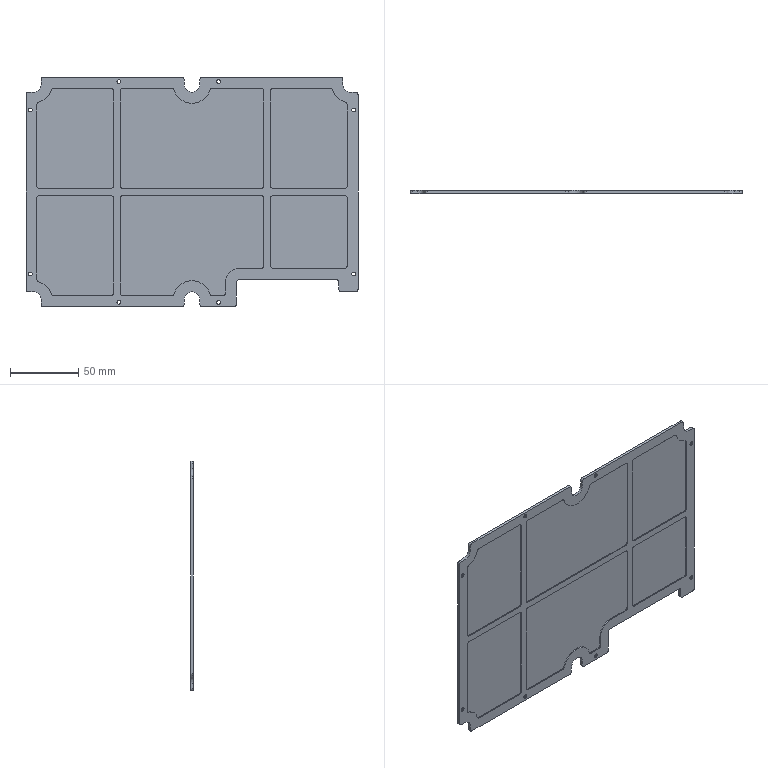CAM job | Mastercam | mm | 7 operations | part box 243 x 2 x 168
1. 2D High Speed (2D Area Mill) | 8 - 8 平铣刀
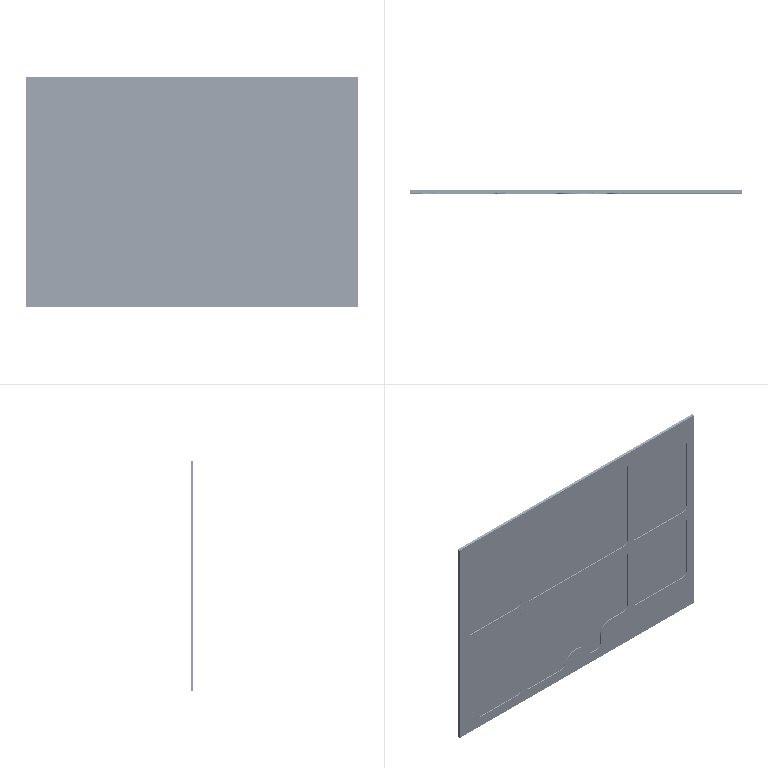2. Contour (2D) | 8 - 8 平铣刀
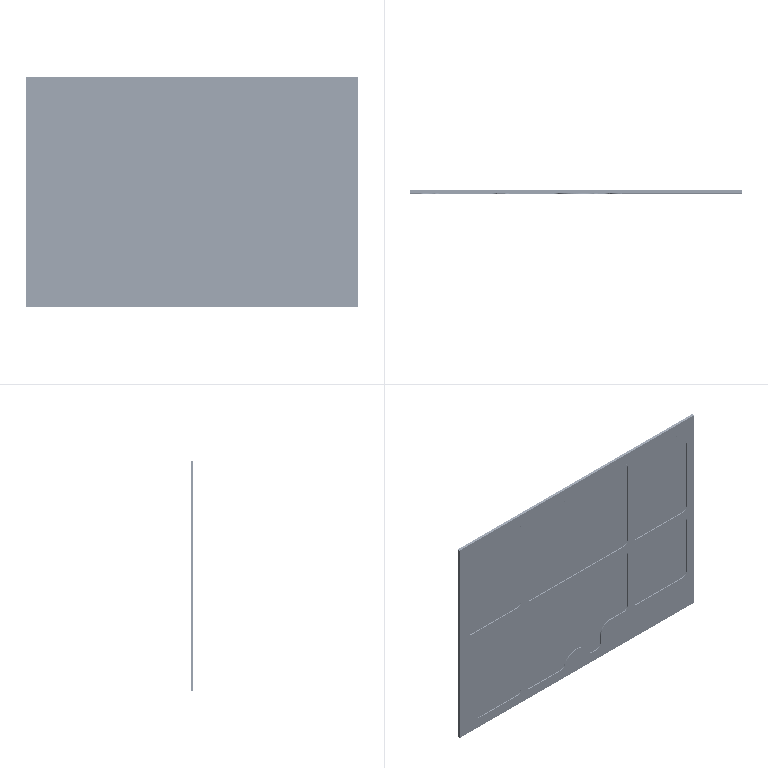3. Contour (Remachining) | 4 - 4 平铣刀
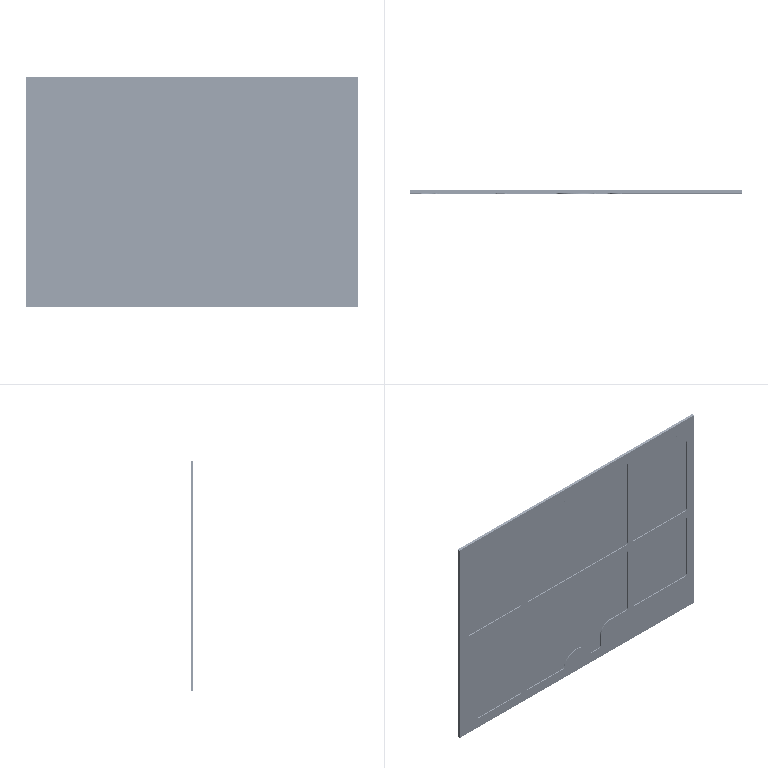4. Contour (Ramp) | 3 - 3 平铣刀
5. Contour (2D chamfer) | 7 - 4 倒角刀
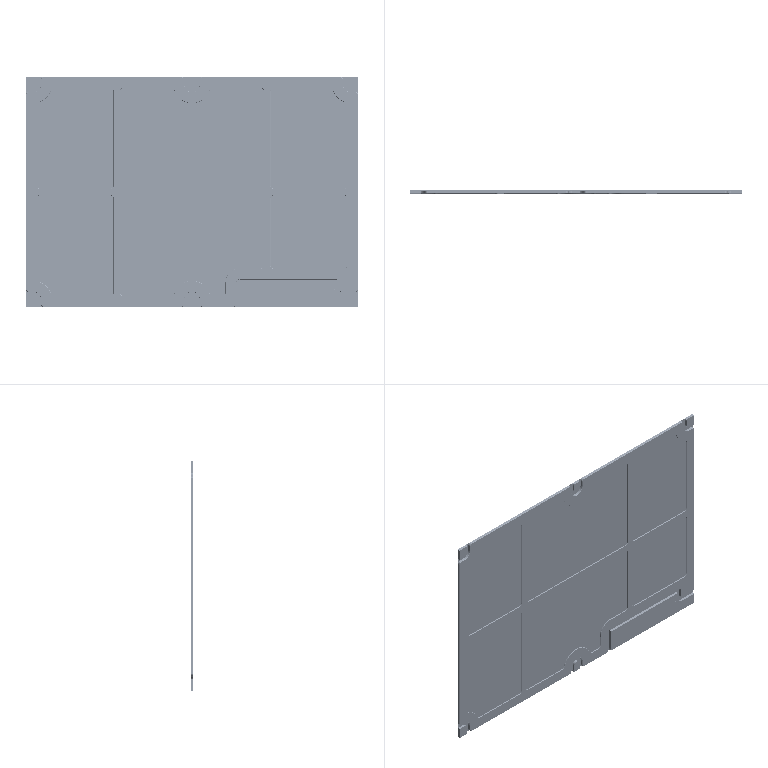6. Drill/Counterbore | 7 - 4 倒角刀
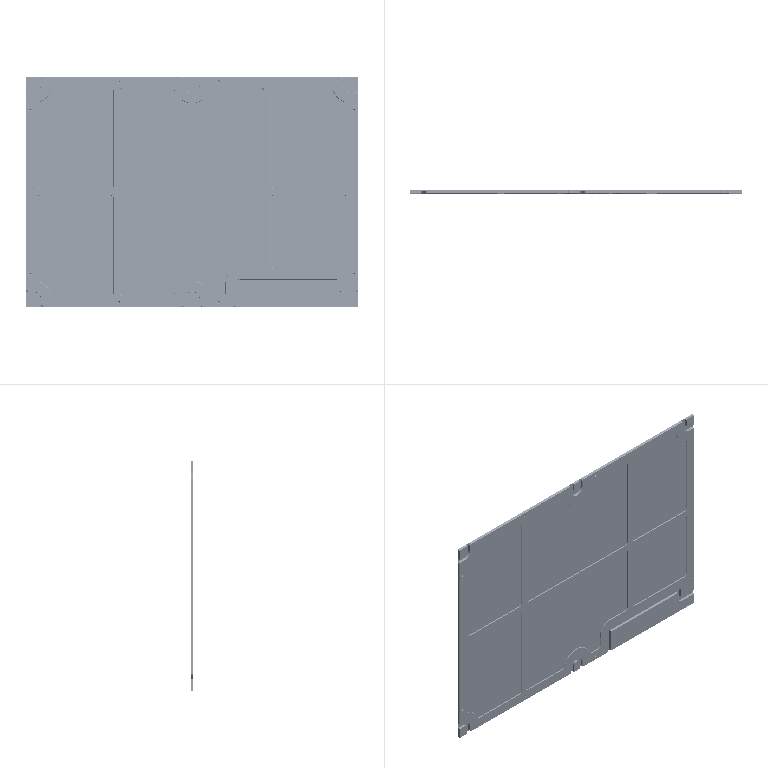7. Contour (2D) | 2 - 2 平铣刀